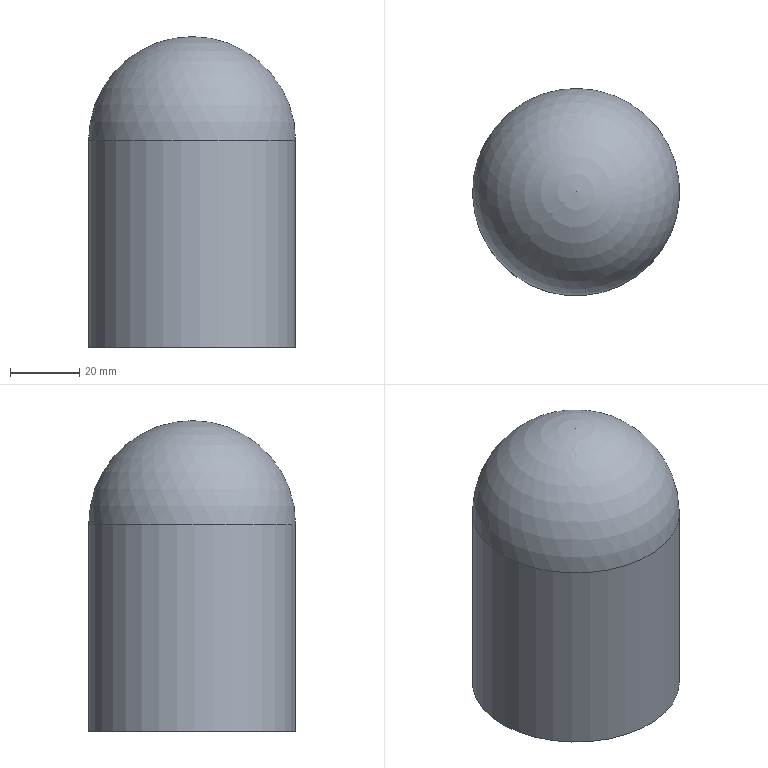Component | NX | SHEJI-WAIGUAN-1 | 1 solid | 6 faces | box 60 x 60 x 90 mm | volume 151936 mm3 | sphere 2 | cylinder 2 | plane 1 | cone 1 | commonest cylinder face diameters 36 x1 60 x1
STEP:
#1=CARTESIAN_POINT('',(0.,0.,0.));
#2=DIRECTION('',(0.,0.,1.));
#3=DIRECTION('',(1.,0.,0.));
#4=AXIS2_PLACEMENT_3D('',#1,#2,#3);
#5=CARTESIAN_POINT('',(6.786,-12.223,116.5));
#6=VERTEX_POINT('',#5);
#7=CARTESIAN_POINT('',(33.214,12.223,116.5));
#8=VERTEX_POINT('',#7);
#9=CARTESIAN_POINT('',(20.,-0.,116.5));
#10=DIRECTION('',(-0.,-0.,1.));
#11=DIRECTION('',(-0.7341,-0.679,-0.));
#12=AXIS2_PLACEMENT_3D('',#9,#10,#11);
#13=CIRCLE('',#12,18.);
#14=CARTESIAN_POINT('',(20.,0.,116.5));
#15=DIRECTION('',(-0.,-0.,1.));
#16=DIRECTION('',(0.7341,0.679,0.));
#17=AXIS2_PLACEMENT_3D('',#14,#15,#16);
#18=SPHERICAL_SURFACE('',#17,18.);
#19=CARTESIAN_POINT('',(3.142,0.));
#20=CARTESIAN_POINT('',(3.237,0.));
#21=CARTESIAN_POINT('',(3.427,0.));
#22=CARTESIAN_POINT('',(3.713,-0.));
#23=CARTESIAN_POINT('',(3.998,0.));
#24=CARTESIAN_POINT('',(4.284,-0.));
#25=CARTESIAN_POINT('',(4.57,0.));
#26=CARTESIAN_POINT('',(4.855,-0.));
#27=CARTESIAN_POINT('',(5.141,0.));
#28=CARTESIAN_POINT('',(5.426,-0.));
#29=CARTESIAN_POINT('',(5.712,0.));
#30=CARTESIAN_POINT('',(5.998,-0.));
#31=CARTESIAN_POINT('',(6.283,0.));
#32=CARTESIAN_POINT('',(6.569,-0.));
#33=CARTESIAN_POINT('',(6.854,0.));
#34=CARTESIAN_POINT('',(7.14,-0.));
#35=CARTESIAN_POINT('',(7.426,0.));
#36=CARTESIAN_POINT('',(7.711,-0.));
#37=CARTESIAN_POINT('',(7.997,0.));
#38=CARTESIAN_POINT('',(8.282,-0.));
#39=CARTESIAN_POINT('',(8.568,0.));
#40=CARTESIAN_POINT('',(8.854,-0.));
#41=CARTESIAN_POINT('',(9.139,0.));
#42=CARTESIAN_POINT('',(9.33,0.));
#43=CARTESIAN_POINT('',(9.425,0.));
#44=B_SPLINE_CURVE_WITH_KNOTS('',3,(#19,#20,#21,#22,#23,#24,#25,#26,#27,#28,#29,#30,#31,#32,#33,#34,#35,#36,#37,#38,#39,#40,#41,#42,#43),.UNSPECIFIED.,.F.,.F.,(4,1,1,1,1,1,1,1,1,1,1,1,1,1,1,1,1,1,1,1,1,1,4),(0.,0.2856,0.5712,0.8568,1.142,1.428,1.714,1.999,2.285,2.57,2.856,3.142,3.427,3.713,3.998,4.284,4.57,4.855,5.141,5.426,5.712,5.998,6.283),.QUASI_UNIFORM_KNOTS.);
#45=(GEOMETRIC_REPRESENTATION_CONTEXT(2)PARAMETRIC_REPRESENTATION_CONTEXT()REPRESENTATION_CONTEXT('',''));
#46=DEFINITIONAL_REPRESENTATION('',(#44),#45);
#47=PCURVE('',#18,#46);
#48=CARTESIAN_POINT('',(20.,0.,56.5));
#49=DIRECTION('',(-0.,-0.,1.));
#50=DIRECTION('',(-0.7341,-0.679,-0.));
#51=AXIS2_PLACEMENT_3D('',#48,#49,#50);
#52=CYLINDRICAL_SURFACE('',#51,18.);
#53=CARTESIAN_POINT('',(0.,60.));
#54=DIRECTION('',(1.,-0.));
#55=VECTOR('',#54,1.);
#56=LINE('',#53,#55);
#57=(GEOMETRIC_REPRESENTATION_CONTEXT(2)PARAMETRIC_REPRESENTATION_CONTEXT()REPRESENTATION_CONTEXT('',''));
#58=DEFINITIONAL_REPRESENTATION('',(#56),#57);
#59=PCURVE('',#52,#58);
#60=SURFACE_CURVE('',#13,(#47,#59),.PCURVE_S1.);
#61=EDGE_CURVE('',#6,#8,#60,.T.);
#62=ORIENTED_EDGE('',*,*,#61,.T.);
#63=CARTESIAN_POINT('',(20.,-0.,134.5));
#64=VERTEX_POINT('',#63);
#65=CARTESIAN_POINT('',(33.214,12.223,116.5));
#66=CARTESIAN_POINT('',(33.214,12.223,120.539));
#67=CARTESIAN_POINT('',(32.437,11.505,124.578));
#68=CARTESIAN_POINT('',(30.885,10.069,128.285));
#69=CARTESIAN_POINT('',(28.652,8.003,131.328));
#70=CARTESIAN_POINT('',(25.93,5.486,133.443));
#71=CARTESIAN_POINT('',(22.965,2.743,134.5));
#72=CARTESIAN_POINT('',(20.,-0.,134.5));
#73=B_SPLINE_CURVE_WITH_KNOTS('',7,(#65,#66,#67,#68,#69,#70,#71,#72),.UNSPECIFIED.,.F.,.F.,(8,8),(0.,1.571),.PIECEWISE_BEZIER_KNOTS.);
#74=CARTESIAN_POINT('',(6.283,0.));
#75=DIRECTION('',(0.,1.));
#76=VECTOR('',#75,1.);
#77=LINE('',#74,#76);
#78=(GEOMETRIC_REPRESENTATION_CONTEXT(2)PARAMETRIC_REPRESENTATION_CONTEXT()REPRESENTATION_CONTEXT('',''));
#79=DEFINITIONAL_REPRESENTATION('',(#77),#78);
#80=PCURVE('',#18,#79);
#81=CARTESIAN_POINT('',(0.,0.));
#82=DIRECTION('',(0.,1.));
#83=VECTOR('',#82,1.);
#84=LINE('',#81,#83);
#85=(GEOMETRIC_REPRESENTATION_CONTEXT(2)PARAMETRIC_REPRESENTATION_CONTEXT()REPRESENTATION_CONTEXT('',''));
#86=DEFINITIONAL_REPRESENTATION('',(#84),#85);
#87=PCURVE('',#18,#86);
#88=SEAM_CURVE('',#73,(#80,#87),.PCURVE_S1.);
#89=EDGE_CURVE('',#8,#64,#88,.T.);
#90=ORIENTED_EDGE('',*,*,#89,.T.);
#91=ORIENTED_EDGE('',*,*,#89,.F.);
#92=CARTESIAN_POINT('',(20.,-0.,116.5));
#93=DIRECTION('',(-0.,-0.,1.));
#94=DIRECTION('',(-0.7341,-0.679,-0.));
#95=AXIS2_PLACEMENT_3D('',#92,#93,#94);
#96=CIRCLE('',#95,18.);
#97=CARTESIAN_POINT('',(-3.142,0.));
#98=CARTESIAN_POINT('',(-3.046,0.));
#99=CARTESIAN_POINT('',(-2.856,0.));
#100=CARTESIAN_POINT('',(-2.57,-0.));
#101=CARTESIAN_POINT('',(-2.285,0.));
#102=CARTESIAN_POINT('',(-1.999,-0.));
#103=CARTESIAN_POINT('',(-1.714,0.));
#104=CARTESIAN_POINT('',(-1.428,-0.));
#105=CARTESIAN_POINT('',(-1.142,0.));
#106=CARTESIAN_POINT('',(-0.8568,-0.));
#107=CARTESIAN_POINT('',(-0.5712,0.));
#108=CARTESIAN_POINT('',(-0.2856,-0.));
#109=CARTESIAN_POINT('',(0.,0.));
#110=CARTESIAN_POINT('',(0.2856,-0.));
#111=CARTESIAN_POINT('',(0.5712,0.));
#112=CARTESIAN_POINT('',(0.8568,-0.));
#113=CARTESIAN_POINT('',(1.142,0.));
#114=CARTESIAN_POINT('',(1.428,-0.));
#115=CARTESIAN_POINT('',(1.714,0.));
#116=CARTESIAN_POINT('',(1.999,-0.));
#117=CARTESIAN_POINT('',(2.285,0.));
#118=CARTESIAN_POINT('',(2.57,-0.));
#119=CARTESIAN_POINT('',(2.856,0.));
#120=CARTESIAN_POINT('',(3.046,0.));
#121=CARTESIAN_POINT('',(3.142,0.));
#122=B_SPLINE_CURVE_WITH_KNOTS('',3,(#97,#98,#99,#100,#101,#102,#103,#104,#105,#106,#107,#108,#109,#110,#111,#112,#113,#114,#115,#116,#117,#118,#119,#120,#121),.UNSPECIFIED.,.F.,.F.,(4,1,1,1,1,1,1,1,1,1,1,1,1,1,1,1,1,1,1,1,1,1,4),(0.,0.2856,0.5712,0.8568,1.142,1.428,1.714,1.999,2.285,2.57,2.856,3.142,3.427,3.713,3.998,4.284,4.57,4.855,5.141,5.426,5.712,5.998,6.283),.QUASI_UNIFORM_KNOTS.);
#123=(GEOMETRIC_REPRESENTATION_CONTEXT(2)PARAMETRIC_REPRESENTATION_CONTEXT()REPRESENTATION_CONTEXT('',''));
#124=DEFINITIONAL_REPRESENTATION('',(#122),#123);
#125=PCURVE('',#18,#124);
#126=CARTESIAN_POINT('',(0.,60.));
#127=DIRECTION('',(1.,0.));
#128=VECTOR('',#127,1.);
#129=LINE('',#126,#128);
#130=(GEOMETRIC_REPRESENTATION_CONTEXT(2)PARAMETRIC_REPRESENTATION_CONTEXT()REPRESENTATION_CONTEXT('',''));
#131=DEFINITIONAL_REPRESENTATION('',(#129),#130);
#132=PCURVE('',#52,#131);
#133=SURFACE_CURVE('',#96,(#125,#132),.PCURVE_S1.);
#134=EDGE_CURVE('',#8,#6,#133,.T.);
#135=ORIENTED_EDGE('',*,*,#134,.T.);
#136=EDGE_LOOP('',(#62,#90,#91,#135));
#137=FACE_BOUND('',#136,.F.);
#138=ADVANCED_FACE('',(#137),#18,.F.);
#139=CARTESIAN_POINT('',(6.786,-12.223,60.5));
#140=VERTEX_POINT('',#139);
#141=CARTESIAN_POINT('',(20.,-0.,60.5));
#142=DIRECTION('',(0.,0.,-1.));
#143=DIRECTION('',(-0.7341,-0.679,-0.));
#144=AXIS2_PLACEMENT_3D('',#141,#142,#143);
#145=CIRCLE('',#144,18.);
#146=CARTESIAN_POINT('',(6.283,4.));
#147=DIRECTION('',(-1.,0.));
#148=VECTOR('',#147,1.);
#149=LINE('',#146,#148);
#150=(GEOMETRIC_REPRESENTATION_CONTEXT(2)PARAMETRIC_REPRESENTATION_CONTEXT()REPRESENTATION_CONTEXT('',''));
#151=DEFINITIONAL_REPRESENTATION('',(#149),#150);
#152=PCURVE('',#52,#151);
#153=CARTESIAN_POINT('',(20.,0.,56.5));
#154=DIRECTION('',(0.,0.,-1.));
#155=DIRECTION('',(0.7341,0.679,0.));
#156=AXIS2_PLACEMENT_3D('',#153,#154,#155);
#157=CONICAL_SURFACE('',#156,22.,0.7854);
#158=CARTESIAN_POINT('',(3.142,-4.));
#159=DIRECTION('',(1.,-0.));
#160=VECTOR('',#159,1.);
#161=LINE('',#158,#160);
#162=(GEOMETRIC_REPRESENTATION_CONTEXT(2)PARAMETRIC_REPRESENTATION_CONTEXT()REPRESENTATION_CONTEXT('',''));
#163=DEFINITIONAL_REPRESENTATION('',(#161),#162);
#164=PCURVE('',#157,#163);
#165=SURFACE_CURVE('',#145,(#152,#164),.PCURVE_S1.);
#166=EDGE_CURVE('',#140,#140,#165,.T.);
#167=ORIENTED_EDGE('',*,*,#166,.F.);
#168=CARTESIAN_POINT('',(6.786,-12.223,60.5));
#169=CARTESIAN_POINT('',(6.786,-12.223,116.5));
#170=B_SPLINE_CURVE_WITH_KNOTS('',1,(#168,#169),.UNSPECIFIED.,.F.,.F.,(2,2),(4.,60.),.PIECEWISE_BEZIER_KNOTS.);
#171=CARTESIAN_POINT('',(6.283,0.));
#172=DIRECTION('',(0.,1.));
#173=VECTOR('',#172,1.);
#174=LINE('',#171,#173);
#175=(GEOMETRIC_REPRESENTATION_CONTEXT(2)PARAMETRIC_REPRESENTATION_CONTEXT()REPRESENTATION_CONTEXT('',''));
#176=DEFINITIONAL_REPRESENTATION('',(#174),#175);
#177=PCURVE('',#52,#176);
#178=CARTESIAN_POINT('',(0.,0.));
#179=DIRECTION('',(0.,1.));
#180=VECTOR('',#179,1.);
#181=LINE('',#178,#180);
#182=(GEOMETRIC_REPRESENTATION_CONTEXT(2)PARAMETRIC_REPRESENTATION_CONTEXT()REPRESENTATION_CONTEXT('',''));
#183=DEFINITIONAL_REPRESENTATION('',(#181),#182);
#184=PCURVE('',#52,#183);
#185=SEAM_CURVE('',#170,(#177,#184),.PCURVE_S1.);
#186=EDGE_CURVE('',#140,#6,#185,.T.);
#187=ORIENTED_EDGE('',*,*,#186,.T.);
#188=ORIENTED_EDGE('',*,*,#134,.F.);
#189=ORIENTED_EDGE('',*,*,#61,.F.);
#190=ORIENTED_EDGE('',*,*,#186,.F.);
#191=EDGE_LOOP('',(#167,#187,#188,#189,#190));
#192=FACE_BOUND('',#191,.F.);
#193=ADVANCED_FACE('',(#192),#52,.F.);
#194=CARTESIAN_POINT('',(3.85,-14.939,56.5));
#195=VERTEX_POINT('',#194);
#196=CARTESIAN_POINT('',(20.,0.,56.5));
#197=DIRECTION('',(-0.,-0.,1.));
#198=DIRECTION('',(-0.7341,-0.679,-0.));
#199=AXIS2_PLACEMENT_3D('',#196,#197,#198);
#200=CIRCLE('',#199,22.);
#201=CARTESIAN_POINT('',(6.786,-12.223,56.5));
#202=DIRECTION('',(-0.,-0.,1.));
#203=DIRECTION('',(-0.7341,-0.679,-0.));
#204=AXIS2_PLACEMENT_3D('',#201,#202,#203);
#205=PLANE('',#204);
#206=CARTESIAN_POINT('',(-18.,0.));
#207=DIRECTION('',(1.,-0.));
#208=AXIS2_PLACEMENT_2D('',#206,#207);
#209=CIRCLE('',#208,22.);
#210=(GEOMETRIC_REPRESENTATION_CONTEXT(2)PARAMETRIC_REPRESENTATION_CONTEXT()REPRESENTATION_CONTEXT('',''));
#211=DEFINITIONAL_REPRESENTATION('',(#209),#210);
#212=PCURVE('',#205,#211);
#213=CARTESIAN_POINT('',(9.425,0.));
#214=DIRECTION('',(-1.,0.));
#215=VECTOR('',#214,1.);
#216=LINE('',#213,#215);
#217=(GEOMETRIC_REPRESENTATION_CONTEXT(2)PARAMETRIC_REPRESENTATION_CONTEXT()REPRESENTATION_CONTEXT('',''));
#218=DEFINITIONAL_REPRESENTATION('',(#216),#217);
#219=PCURVE('',#157,#218);
#220=SURFACE_CURVE('',#200,(#212,#219),.PCURVE_S1.);
#221=EDGE_CURVE('',#195,#195,#220,.T.);
#222=ORIENTED_EDGE('',*,*,#221,.T.);
#223=EDGE_LOOP('',(#222));
#224=FACE_BOUND('',#223,.T.);
#225=CARTESIAN_POINT('',(-2.023,-20.371,56.5));
#226=VERTEX_POINT('',#225);
#227=CARTESIAN_POINT('',(20.,0.,56.5));
#228=DIRECTION('',(-0.,-0.,1.));
#229=DIRECTION('',(-0.7341,-0.679,-0.));
#230=AXIS2_PLACEMENT_3D('',#227,#228,#229);
#231=CIRCLE('',#230,30.);
#232=CARTESIAN_POINT('',(-18.,0.));
#233=DIRECTION('',(1.,-0.));
#234=AXIS2_PLACEMENT_2D('',#232,#233);
#235=CIRCLE('',#234,30.);
#236=(GEOMETRIC_REPRESENTATION_CONTEXT(2)PARAMETRIC_REPRESENTATION_CONTEXT()REPRESENTATION_CONTEXT('',''));
#237=DEFINITIONAL_REPRESENTATION('',(#235),#236);
#238=PCURVE('',#205,#237);
#239=CARTESIAN_POINT('',(20.,0.,56.5));
#240=DIRECTION('',(-0.,-0.,1.));
#241=DIRECTION('',(-0.7341,-0.679,-0.));
#242=AXIS2_PLACEMENT_3D('',#239,#240,#241);
#243=CYLINDRICAL_SURFACE('',#242,30.);
#244=CARTESIAN_POINT('',(0.,0.));
#245=DIRECTION('',(1.,0.));
#246=VECTOR('',#245,1.);
#247=LINE('',#244,#246);
#248=(GEOMETRIC_REPRESENTATION_CONTEXT(2)PARAMETRIC_REPRESENTATION_CONTEXT()REPRESENTATION_CONTEXT('',''));
#249=DEFINITIONAL_REPRESENTATION('',(#247),#248);
#250=PCURVE('',#243,#249);
#251=SURFACE_CURVE('',#231,(#238,#250),.PCURVE_S1.);
#252=EDGE_CURVE('',#226,#226,#251,.T.);
#253=ORIENTED_EDGE('',*,*,#252,.F.);
#254=EDGE_LOOP('',(#253));
#255=FACE_BOUND('',#254,.T.);
#256=ADVANCED_FACE('',(#224,#255),#205,.F.);
#257=CARTESIAN_POINT('',(-2.023,-20.371,116.5));
#258=VERTEX_POINT('',#257);
#259=CARTESIAN_POINT('',(20.,-0.,116.5));
#260=DIRECTION('',(-0.,-0.,1.));
#261=DIRECTION('',(-0.7341,-0.679,-0.));
#262=AXIS2_PLACEMENT_3D('',#259,#260,#261);
#263=CIRCLE('',#262,30.);
#264=CARTESIAN_POINT('',(0.,60.));
#265=DIRECTION('',(1.,0.));
#266=VECTOR('',#265,1.);
#267=LINE('',#264,#266);
#268=(GEOMETRIC_REPRESENTATION_CONTEXT(2)PARAMETRIC_REPRESENTATION_CONTEXT()REPRESENTATION_CONTEXT('',''));
#269=DEFINITIONAL_REPRESENTATION('',(#267),#268);
#270=PCURVE('',#243,#269);
#271=CARTESIAN_POINT('',(20.,0.,116.5));
#272=DIRECTION('',(-0.,-0.,1.));
#273=DIRECTION('',(-0.7341,-0.679,-0.));
#274=AXIS2_PLACEMENT_3D('',#271,#272,#273);
#275=SPHERICAL_SURFACE('',#274,30.);
#276=CARTESIAN_POINT('',(-0.,0.));
#277=CARTESIAN_POINT('',(0.0952,-0.));
#278=CARTESIAN_POINT('',(0.2856,-0.));
#279=CARTESIAN_POINT('',(0.5712,0.));
#280=CARTESIAN_POINT('',(0.8568,-0.));
#281=CARTESIAN_POINT('',(1.142,0.));
#282=CARTESIAN_POINT('',(1.428,0.));
#283=CARTESIAN_POINT('',(1.714,-0.));
#284=CARTESIAN_POINT('',(1.999,0.));
#285=CARTESIAN_POINT('',(2.285,0.));
#286=CARTESIAN_POINT('',(2.57,-0.));
#287=CARTESIAN_POINT('',(2.856,-0.));
#288=CARTESIAN_POINT('',(3.142,-0.));
#289=CARTESIAN_POINT('',(3.427,-0.));
#290=CARTESIAN_POINT('',(3.713,-0.));
#291=CARTESIAN_POINT('',(3.998,0.));
#292=CARTESIAN_POINT('',(4.284,0.));
#293=CARTESIAN_POINT('',(4.57,-0.));
#294=CARTESIAN_POINT('',(4.855,0.));
#295=CARTESIAN_POINT('',(5.141,0.));
#296=CARTESIAN_POINT('',(5.426,-0.));
#297=CARTESIAN_POINT('',(5.712,0.));
#298=CARTESIAN_POINT('',(5.998,-0.));
#299=CARTESIAN_POINT('',(6.188,-0.));
#300=CARTESIAN_POINT('',(6.283,0.));
#301=B_SPLINE_CURVE_WITH_KNOTS('',3,(#276,#277,#278,#279,#280,#281,#282,#283,#284,#285,#286,#287,#288,#289,#290,#291,#292,#293,#294,#295,#296,#297,#298,#299,#300),.UNSPECIFIED.,.F.,.F.,(4,1,1,1,1,1,1,1,1,1,1,1,1,1,1,1,1,1,1,1,1,1,4),(0.,0.2856,0.5712,0.8568,1.142,1.428,1.714,1.999,2.285,2.57,2.856,3.142,3.427,3.713,3.998,4.284,4.57,4.855,5.141,5.426,5.712,5.998,6.283),.QUASI_UNIFORM_KNOTS.);
#302=(GEOMETRIC_REPRESENTATION_CONTEXT(2)PARAMETRIC_REPRESENTATION_CONTEXT()REPRESENTATION_CONTEXT('',''));
#303=DEFINITIONAL_REPRESENTATION('',(#301),#302);
#304=PCURVE('',#275,#303);
#305=SURFACE_CURVE('',#263,(#270,#304),.PCURVE_S1.);
#306=EDGE_CURVE('',#258,#258,#305,.T.);
#307=ORIENTED_EDGE('',*,*,#306,.F.);
#308=CARTESIAN_POINT('',(-2.023,-20.371,56.5));
#309=CARTESIAN_POINT('',(-2.023,-20.371,116.5));
#310=B_SPLINE_CURVE_WITH_KNOTS('',1,(#308,#309),.UNSPECIFIED.,.F.,.F.,(2,2),(0.,60.),.PIECEWISE_BEZIER_KNOTS.);
#311=CARTESIAN_POINT('',(0.,0.));
#312=DIRECTION('',(0.,1.));
#313=VECTOR('',#312,1.);
#314=LINE('',#311,#313);
#315=(GEOMETRIC_REPRESENTATION_CONTEXT(2)PARAMETRIC_REPRESENTATION_CONTEXT()REPRESENTATION_CONTEXT('',''));
#316=DEFINITIONAL_REPRESENTATION('',(#314),#315);
#317=PCURVE('',#243,#316);
#318=CARTESIAN_POINT('',(6.283,0.));
#319=DIRECTION('',(0.,1.));
#320=VECTOR('',#319,1.);
#321=LINE('',#318,#320);
#322=(GEOMETRIC_REPRESENTATION_CONTEXT(2)PARAMETRIC_REPRESENTATION_CONTEXT()REPRESENTATION_CONTEXT('',''));
#323=DEFINITIONAL_REPRESENTATION('',(#321),#322);
#324=PCURVE('',#243,#323);
#325=SEAM_CURVE('',#310,(#317,#324),.PCURVE_S1.);
#326=EDGE_CURVE('',#226,#258,#325,.T.);
#327=ORIENTED_EDGE('',*,*,#326,.F.);
#328=ORIENTED_EDGE('',*,*,#252,.T.);
#329=ORIENTED_EDGE('',*,*,#326,.T.);
#330=EDGE_LOOP('',(#307,#327,#328,#329));
#331=FACE_BOUND('',#330,.T.);
#332=ADVANCED_FACE('',(#331),#243,.T.);
#333=ORIENTED_EDGE('',*,*,#306,.T.);
#334=CARTESIAN_POINT('',(20.,-0.,146.5));
#335=VERTEX_POINT('',#334);
#336=CARTESIAN_POINT('',(-2.023,-20.371,116.5));
#337=CARTESIAN_POINT('',(-2.023,-20.371,123.232));
#338=CARTESIAN_POINT('',(-0.729,-19.175,129.964));
#339=CARTESIAN_POINT('',(1.858,-16.781,136.142));
#340=CARTESIAN_POINT('',(5.581,-13.338,141.213));
#341=CARTESIAN_POINT('',(10.116,-9.143,144.738));
#342=CARTESIAN_POINT('',(15.058,-4.571,146.5));
#343=CARTESIAN_POINT('',(20.,-0.,146.5));
#344=B_SPLINE_CURVE_WITH_KNOTS('',7,(#336,#337,#338,#339,#340,#341,#342,#343),.UNSPECIFIED.,.F.,.F.,(8,8),(0.,1.571),.PIECEWISE_BEZIER_KNOTS.);
#345=CARTESIAN_POINT('',(6.283,0.));
#346=DIRECTION('',(0.,1.));
#347=VECTOR('',#346,1.);
#348=LINE('',#345,#347);
#349=(GEOMETRIC_REPRESENTATION_CONTEXT(2)PARAMETRIC_REPRESENTATION_CONTEXT()REPRESENTATION_CONTEXT('',''));
#350=DEFINITIONAL_REPRESENTATION('',(#348),#349);
#351=PCURVE('',#275,#350);
#352=CARTESIAN_POINT('',(-0.,0.));
#353=DIRECTION('',(0.,1.));
#354=VECTOR('',#353,1.);
#355=LINE('',#352,#354);
#356=(GEOMETRIC_REPRESENTATION_CONTEXT(2)PARAMETRIC_REPRESENTATION_CONTEXT()REPRESENTATION_CONTEXT('',''));
#357=DEFINITIONAL_REPRESENTATION('',(#355),#356);
#358=PCURVE('',#275,#357);
#359=SEAM_CURVE('',#344,(#351,#358),.PCURVE_S1.);
#360=EDGE_CURVE('',#258,#335,#359,.T.);
#361=ORIENTED_EDGE('',*,*,#360,.T.);
#362=ORIENTED_EDGE('',*,*,#360,.F.);
#363=EDGE_LOOP('',(#333,#361,#362));
#364=FACE_BOUND('',#363,.T.);
#365=ADVANCED_FACE('',(#364),#275,.T.);
#366=ORIENTED_EDGE('',*,*,#166,.T.);
#367=CARTESIAN_POINT('',(6.786,-12.223,60.5));
#368=CARTESIAN_POINT('',(3.85,-14.939,56.5));
#369=B_SPLINE_CURVE_WITH_KNOTS('',1,(#367,#368),.UNSPECIFIED.,.F.,.F.,(2,2),(-5.657,0.),.PIECEWISE_BEZIER_KNOTS.);
#370=CARTESIAN_POINT('',(9.425,0.));
#371=DIRECTION('',(0.,1.));
#372=VECTOR('',#371,1.);
#373=LINE('',#370,#372);
#374=(GEOMETRIC_REPRESENTATION_CONTEXT(2)PARAMETRIC_REPRESENTATION_CONTEXT()REPRESENTATION_CONTEXT('',''));
#375=DEFINITIONAL_REPRESENTATION('',(#373),#374);
#376=PCURVE('',#157,#375);
#377=CARTESIAN_POINT('',(3.142,0.));
#378=DIRECTION('',(0.,1.));
#379=VECTOR('',#378,1.);
#380=LINE('',#377,#379);
#381=(GEOMETRIC_REPRESENTATION_CONTEXT(2)PARAMETRIC_REPRESENTATION_CONTEXT()REPRESENTATION_CONTEXT('',''));
#382=DEFINITIONAL_REPRESENTATION('',(#380),#381);
#383=PCURVE('',#157,#382);
#384=SEAM_CURVE('',#369,(#376,#383),.PCURVE_S1.);
#385=EDGE_CURVE('',#140,#195,#384,.T.);
#386=ORIENTED_EDGE('',*,*,#385,.T.);
#387=ORIENTED_EDGE('',*,*,#221,.T.);
#388=ORIENTED_EDGE('',*,*,#385,.F.);
#389=EDGE_LOOP('',(#366,#386,#387,#388));
#390=FACE_BOUND('',#389,.F.);
#391=ADVANCED_FACE('',(#390),#157,.F.);
#392=CLOSED_SHELL('',(#138,#193,#256,#332,#365,#391));
#393=MANIFOLD_SOLID_BREP('',#392);
#394=(LENGTH_UNIT()NAMED_UNIT(*)SI_UNIT(.MILLI.,.METRE.));
#395=UNCERTAINTY_MEASURE_WITH_UNIT(LENGTH_MEASURE(0.00001),#394,'','');
#396=(NAMED_UNIT(*)PLANE_ANGLE_UNIT()SI_UNIT($,.RADIAN.));
#397=(NAMED_UNIT(*)SI_UNIT($,.STERADIAN.)SOLID_ANGLE_UNIT());
#398=(GEOMETRIC_REPRESENTATION_CONTEXT(3)GLOBAL_UNCERTAINTY_ASSIGNED_CONTEXT((#395))GLOBAL_UNIT_ASSIGNED_CONTEXT((#394,#396,#397))REPRESENTATION_CONTEXT('',''));
#399=ADVANCED_BREP_SHAPE_REPRESENTATION('',(#4,#393),#398);